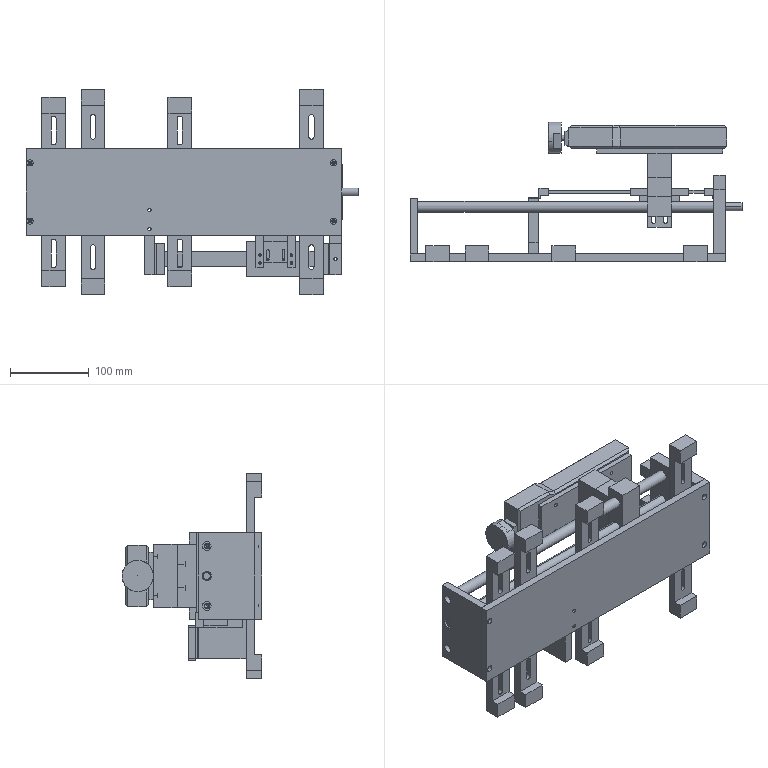Assembly | SolidWorks | mm | 24 component files | 24 solids | 580 faces | box 421 x 177.5 x 260 mm | volume 1942714 mm3 | plane 262 | cylinder 230 | cone 88 | commonest cylinder face diameters 4.2 x44 5.5 x32 3.3 x28 4.5 x20 6.5 x16 10 x12 14 x12 5 x12
Bill of materials:
CS021-A10-A001 | 1 | AL6061 | Thin, long rectangular flat plate with four small holes near the corners and two smaller holes in a vertical pair, a little left of center.
CS021-A10-A002 | 1 | 45 | Thick rectangular plate with two rectangular tabs sticking out from one edge, one round through hole off-center, and two small holes on the opposite narrow edge face.
CS021-A10-A003 | 1 | AL6061 | Thick rectangular plate with three through holes in a line near one long edge (a larger middle hole between two smaller ones) and two small holes on the opposite narrow edge face.
CS021-A10-A005 | 1 | Q235 | Long rectangular block with three equally spaced round holes in a line, going through the block between two opposite side faces.
CS021-A10-A006 | 2 | AL6061 | Long slender cylindrical rod with a small hole along its axis at the visible end.
CS021-A10-A007 | 1 | AL6061 | Thin rectangular plate with eight through holes: four smaller holes in a rectangular pattern toward the ends and four larger holes in a central square-like group.
CS021-A10-A008 | 1 | SUS304 | Short cylindrical disc with a small central hole and a flat cut along one side that covers most of the disc's thickness, leaving a thin full-diameter rim at one end.
CS021-A10-A009 | 1 | AL6061 | Rectangular block with four round holes on one face in a rectangular pattern, two near each end, going through the block.
CS021-A10-A012 | 4 | AL6061 | Block with an L-shaped side profile: a thin upright plate with a thicker lip along one end, and an elongated slot through the thin section.
CS021-A10-A022 | 2 | AL6061 | Long thin bar with a C-shaped (channel) side profile, with short lips at both ends on the same side, and two long slots through the main web.
CS021-A10-A024 | 2 | AL6061 | Long bar with a square cross-section: two through holes near one end go through one way, and a single through hole near the other end goes through at right angles to them.
CS021-A10-A025 | 1 | AL6061 | L-shaped bracket of rectangular section, with two through holes in the horizontal leg and one hole in the vertical leg at right angles to them.
CS021-A10-A026 | 1 | AL6061 | Thick, flat plate with an L-shaped outline: a narrow tall upright leg joined to a wider, shorter base section. Two round holes pass through the narrow upright leg.
CS021-A10-A027 | 1 | AL6061 | Rectangular prism block, taller than it is wide, with four round holes in a 2x2 pattern on one long face.
CS021-A10-A028 | 1 | AL6061 | Angle bracket: two flat legs of roughly equal thickness joined at a right angle. Each leg has two parallel, round-ended slots.
CS021-DigitalPush-PullForceGaugeSF-500 | 1 | POM (White) | Long rectangular box-like body with chamfered long edges and a shallow step/taper in width near one end. A small tapered boss with a protruding cylindrical pin sits on the end face. Four small holes are on one large face.
CS021-DigitalScale-Range100 | 1 | AL6061 | Long, slender bar-like part with a wider rectangular centre block carrying a pattern of small holes, narrower bar sections on either side, and stepped end pads ending in plate-like end tabs. Each end tab has a round-ended slot.
CS021-T-BallScrew16x4(ZYCS002) | 1 | 45 | Long, slender stepped cylindrical shaft/rod: a long main diameter with a short reduced-diameter stub at one end and a longer reduced-diameter section at the other end.
Mates:
1. distance | CS021-A10-A008-1 face at (27.448, 172.317, 0) dir (1, 0, 0) | CS021-DigitalPush-PullForceGaugeSF-500-2 face at (17.448, 172.317, 0) dir (-1, 0, 0)
2. concentric | CS021-DigitalPush-PullForceGaugeSF-500-2 face at (17.448, 172.317, 0) dir (1, 0, 0) r 3 | CS021-A10-A008-1 face at (27.448, 172.317, 0) dir (-1, 0, 0) r 20
3. coincident | CS021-A10-A012-2 face at (-64.051, 35.017, 130) dir (0, 1, 0) | CS021-A10-A012-3 face at (212.949, 35.017, 130) dir (0, 1, 0)
4. coincident | CS021-A10-A012-2 face at (-64.051, 15.017, 130) dir (0, 0, 1) | CS021-A10-A012-3 face at (212.949, 15.017, 130) dir (0, 0, 1)
5. coincident | CS021-A10-A001-1 face at (35.949, 24.817, 0) dir (0, 1, 0) | CS021-A10-A012-3 face at (212.949, 24.817, 40) dir (0, -1, 0)
6. distance | CS021-A10-A012-3 face at (212.949, 35.017, 40) dir (0, 0, -1) | CS021-A10-A001-1 face at (-164.051, 24.817, 55) dir (0, 0, 1)
7. distance | CS021-A10-A012-2 face at (-94.051, 15.017, 130) dir (-1, 0, 0) | CS021-A10-A001-1 face at (-164.051, 24.817, 55) dir (-1, 0, 0)
8. coincident | CS021-A10-A001-1 face at (35.949, 24.817, 0) dir (0, 1, 0) | CS021-A10-A003-1 face at (-164.051, 24.817, -55) dir (0, -1, 0)
9. coincident | CS021-A10-A001-1 face at (-164.051, 24.817, 55) dir (-1, 0, 0) | CS021-A10-A003-1 face at (-164.051, 59.817, 0) dir (-1, 0, 0)
10. coincident | CS021-A10-A001-1 face at (-164.051, 24.817, -55) dir (0, 0, -1) | CS021-A10-A003-1 face at (-164.051, 24.817, -55) dir (0, 0, -1)
11. concentric | CS021-A10-A003-1 face at (-164.051, 84.817, -38) dir (-1, 0, 0) r 3.3 | CS021-A10-A006-1 face at (-154.051, 84.817, -38) dir (1, 0, 0) r 7
12. coincident | CS021-A10-A003-1 face at (-154.051, 59.817, 0) dir (1, 0, 0) | CS021-A10-A006-1 face at (-154.051, 84.817, -38) dir (-1, 0, 0)
13. concentric | CS021-A10-A003-1 face at (-164.051, 84.817, 38) dir (-1, 0, 0) r 3.3 | CS021-A10-A006-2 face at (-154.051, 84.817, 38) dir (1, 0, 0) r 7
14. coincident | CS021-A10-A003-1 face at (-154.051, 59.817, 0) dir (1, 0, 0) | CS021-A10-A006-2 face at (-154.051, 84.817, 38) dir (-1, 0, 0)
15. concentric | CS021-A10-A003-1 face at (-159.051, 84.817, 0) dir (1, 0, 0) r 8 | CS021-T-BallScrew16x4(ZYCS002)-1 face at (220.949, 84.817, 0) dir (-1, 0, 0) r 7
16. coincident | CS021-A10-A003-1 face at (-154.051, 59.817, 0) dir (1, 0, 0) | CS021-T-BallScrew16x4(ZYCS002)-1 face at (-154.051, 84.817, 0) dir (-1, 0, 0)
17. concentric | CS021-T-BallScrew16x4(ZYCS002)-1 face at (220.949, 84.817, 0) dir (-1, 0, 0) r 7 | CS021-A10-A005-3 face at (137.449, 84.817, 0) dir (1, 0, 0) r 7
18. parallel | CS021-A10-A003-1 face at (-164.051, 94.817, -55) dir (0, 1, 0) | CS021-A10-A005-3 face at (167.449, 97.317, 55) dir (0, 1, 0)
19. distance | CS021-A10-A007-1 face at (152.449, 152.317, 0) dir (0, -1, 0) | CS021-A10-A005-3 face at (167.449, 97.317, 55) dir (0, 1, 0)
20. concentric | CS021-A10-A007-1 face at (162.449, 158.317, 15) dir (0, 1, 0) r 2.75 | CS021-A10-A005-3 face at (162.449, 97.317, 15) dir (0, 1, 0) r 2.1
21. concentric | CS021-A10-A007-1 face at (142.449, 158.317, -15) dir (0, 1, 0) r 2.75 | CS021-A10-A005-3 face at (142.449, 97.317, -15) dir (0, 1, 0) r 2.1
22. concentric | CS021-DigitalPush-PullForceGaugeSF-500-2 face at (197.448, 158.317, -20) dir (0, -1, 0) r 1.65 | CS021-A10-A007-1 face at (197.448, 158.317, -20) dir (0, 1, 0) r 2.25
23. concentric | CS021-DigitalPush-PullForceGaugeSF-500-2 face at (197.448, 158.317, 20) dir (0, -1, 0) r 1.65 | CS021-A10-A007-1 face at (197.448, 158.317, 20) dir (0, 1, 0) r 2.25
24. coincident | CS021-DigitalPush-PullForceGaugeSF-500-2 face at (237.448, 158.317, 0) dir (0, -1, 0) | CS021-A10-A007-1 face at (152.449, 158.317, 0) dir (0, 1, 0)
25. coincident | CS021-A10-A001-1 face at (35.949, 24.817, 0) dir (0, 1, 0) | CS021-A10-A002-1 face at (220.949, 24.817, -55) dir (0, -1, 0)
26. coincident | CS021-A10-A001-1 face at (235.949, 24.817, 55) dir (1, 0, 0) | CS021-A10-A002-1 face at (235.949, 74.817, 0) dir (1, 0, 0)
27. coincident | CS021-A10-A001-1 face at (-164.051, 24.817, 55) dir (0, 0, 1) | CS021-A10-A002-1 face at (220.949, 24.817, 55) dir (0, 0, 1)
28. distance | CS021-A10-A005-3 face at (167.449, 97.317, 55) dir (0, 1, 0) | CS021-A10-A009-1 face at (152.449, 122.317, 0) dir (0, -1, 0)
29. width | CS021-A10-A005-3 face at (137.449, 84.817, 0) dir (-1, 0, 0) | CS021-A10-A005-3 face at (167.449, 84.817, 0) dir (1, 0, 0) | CS021-A10-A009-1 face at (167.449, 122.317, 40) dir (1, 0, 0) | CS021-A10-A009-1 face at (137.449, 122.317, 40) dir (-1, 0, 0)
30. width | CS021-A10-A005-3 face at (167.449, 72.317, 55) dir (0, 0, 1) | CS021-A10-A005-3 face at (167.449, 72.317, -55) dir (0, 0, -1) | CS021-A10-A009-1 face at (167.449, 122.317, 40) dir (0, 0, 1) | CS021-A10-A009-1 face at (167.449, 122.317, -40) dir (0, 0, -1)
31. distance | CS021-DigitalScale-Range100-1 face at (0.9486, 94.817, -105) dir (0, -1, 0) | CS021-A10-A001-1 face at (35.949, 24.817, 0) dir (0, 1, 0)
32. distance | CS021-DigitalScale-Range100-1 face at (110.449, 103.817, -105) dir (0, 0, -1) | CS021-A10-A003-1 face at (-164.051, 24.817, -55) dir (0, 0, -1)
33. coincident | CS021-A10-A001-1 face at (35.949, 24.817, 0) dir (0, 1, 0) | CS021-A10-A022-1 face at (-144.051, 24.817, 100) dir (0, -1, 0)
34. coincident | CS021-A10-A001-1 face at (35.949, 24.817, 0) dir (0, 1, 0) | CS021-A10-A022-1 face at (-144.051, 24.817, 100) dir (0, -1, 0)
35. distance | CS021-A10-A003-1 face at (-154.051, 59.817, 0) dir (1, 0, 0) | CS021-A10-A022-1 face at (-144.051, 15.017, 0) dir (-1, 0, 0)
36. width | CS021-A10-A022-1 face at (-144.051, 15.017, 120) dir (0, 0, 1) | CS021-A10-A022-1 face at (-144.051, 15.017, -120) dir (0, 0, -1) | CS021-A10-A001-1 face at (-164.051, 24.817, 55) dir (0, 0, 1) | CS021-A10-A001-1 face at (-164.051, 24.817, -55) dir (0, 0, -1)
37. coincident | CS021-A10-A022-1 face at (-144.051, 35.017, -120) dir (0, 1, 0) | CS021-A10-A022-2 face at (15.949, 35.017, -120) dir (0, 1, 0)
38. coincident | CS021-A10-A022-1 face at (-144.051, 15.017, 120) dir (0, 0, 1) | CS021-A10-A022-2 face at (15.949, 15.017, 120) dir (0, 0, 1)
39. distance | CS021-A10-A022-1 face at (-144.051, 15.017, 0) dir (-1, 0, 0) | CS021-A10-A022-2 face at (15.949, 15.017, 0) dir (-1, 0, 0)
40. concentric | CS021-DigitalScale-Range100-1 face at (172.449, 98.817, -90) dir (0, -1, 0) r 1.25 | CS021-A10-A024-1 face at (172.449, 98.817, -90) dir (0, 1, 0) r 1.65
41. concentric | CS021-DigitalScale-Range100-1 face at (172.449, 98.817, -80) dir (0, -1, 0) r 1.25 | CS021-A10-A024-1 face at (172.449, 98.817, -80) dir (0, 1, 0) r 1.65
42. coincident | CS021-DigitalScale-Range100-1 face at (110.449, 98.817, -85) dir (0, -1, 0) | CS021-A10-A024-1 face at (177.449, 98.817, -46) dir (0, 1, 0)
43. concentric | CS021-DigitalScale-Range100-1 face at (132.449, 98.817, -90) dir (0, -1, 0) r 1.25 | CS021-A10-A024-2 face at (132.449, 98.817, -90) dir (0, 1, 0) r 1.65
44. concentric | CS021-DigitalScale-Range100-1 face at (132.449, 98.817, -80) dir (0, -1, 0) r 1.25 | CS021-A10-A024-2 face at (132.449, 98.817, -80) dir (0, 1, 0) r 1.65
45. coincident | CS021-DigitalScale-Range100-1 face at (110.449, 98.817, -85) dir (0, -1, 0) | CS021-A10-A024-2 face at (137.449, 98.817, -46) dir (0, 1, 0)
46. distance | CS021-DigitalScale-Range100-1 face at (234.449, 94.817, -105) dir (1, 0, 0) | CS021-A10-A002-1 face at (235.949, 74.817, 0) dir (1, 0, 0)
47. coincident | CS021-A10-A002-1 face at (235.949, 74.817, 0) dir (1, 0, 0) | CS021-A10-A025-1 face at (235.949, 29.817, -55) dir (1, 0, 0)
48. coincident | CS021-A10-A002-1 face at (220.949, 24.817, -55) dir (0, 0, -1) | CS021-A10-A025-1 face at (235.949, 29.817, -55) dir (0, 0, 1)
49. coincident | CS021-DigitalScale-Range100-1 face at (219.949, 94.817, -105) dir (0, -1, 0) | CS021-A10-A025-1 face at (235.949, 94.817, -55) dir (0, 1, 0)
50. coincident | CS021-DigitalScale-Range100-1 face at (110.449, 103.817, -105) dir (0, 0, -1) | CS021-A10-A026-1 face at (-1.551, 29.817, -105) dir (0, 0, -1)
51. coincident | CS021-DigitalScale-Range100-1 face at (0.9486, 94.817, -105) dir (0, -1, 0) | CS021-A10-A026-1 face at (-1.551, 94.817, -65) dir (0, 1, 0)
52. coincident | CS021-DigitalScale-Range100-1 face at (-13.551, 94.817, -105) dir (-1, 0, 0) | CS021-A10-A026-1 face at (-13.551, 29.817, -65) dir (-1, 0, 0)
53. coincident | CS021-A10-A005-3 face at (167.449, 97.317, 55) dir (0, 1, 0) | CS021-A10-A027-1 face at (152.449, 97.317, 0) dir (0, -1, 0)
54. coincident | CS021-A10-A009-1 face at (137.449, 122.317, 40) dir (-1, 0, 0) | CS021-A10-A027-1 face at (137.449, 97.317, -40) dir (-1, 0, 0)
55. coincident | CS021-A10-A009-1 face at (167.449, 122.317, -40) dir (0, 0, -1) | CS021-A10-A027-1 face at (137.449, 97.317, -40) dir (0, 0, -1)
56. coincident | CS021-A10-A005-3 face at (167.449, 72.317, -55) dir (0, 0, -1) | CS021-A10-A028-1 face at (167.449, 98.817, -55) dir (0, 0, 1)
57. coincident | CS021-DigitalScale-Range100-1 face at (110.449, 98.817, -85) dir (0, -1, 0) | CS021-A10-A028-1 face at (167.449, 98.817, -90) dir (0, 1, 0)
58. width | CS021-A10-A028-1 face at (137.449, 58.817, -55) dir (-1, 0, 0) | CS021-A10-A028-1 face at (167.449, 58.817, -55) dir (1, 0, 0) | CS021-A10-A005-3 face at (137.449, 84.817, 0) dir (-1, 0, 0) | CS021-A10-A005-3 face at (167.449, 84.817, 0) dir (1, 0, 0)